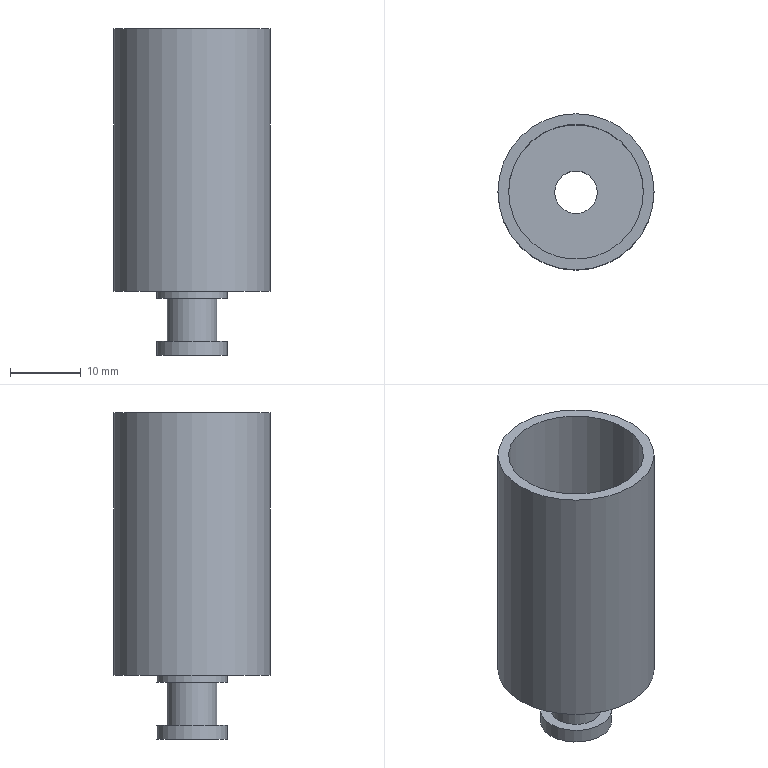Component | NX | PUMP_FLANGE_FITTING | 1 solid | 12 faces | box 22 x 22 x 46 mm | volume 4552 mm3 | plane 6 | cylinder 6 | commonest cylinder face diameters 10 x2 6 x1 7 x1 22 x1 19 x1
STEP:
#1=CARTESIAN_POINT('',(0.,0.,0.));
#2=DIRECTION('',(0.,0.,1.));
#3=DIRECTION('',(1.,0.,0.));
#4=AXIS2_PLACEMENT_3D('',#1,#2,#3);
#5=CARTESIAN_POINT('',(-2.267,-0.01624,77.));
#6=VERTEX_POINT('',#5);
#7=CARTESIAN_POINT('',(-5.267,-0.01624,77.));
#8=DIRECTION('',(0.,0.,1.));
#9=DIRECTION('',(1.,0.,0.));
#10=AXIS2_PLACEMENT_3D('',#7,#8,#9);
#11=CIRCLE('',#10,3.);
#12=CARTESIAN_POINT('',(-5.267,-0.01624,77.));
#13=DIRECTION('',(0.,0.,1.));
#14=DIRECTION('',(1.,0.,0.));
#15=AXIS2_PLACEMENT_3D('',#12,#13,#14);
#16=PLANE('',#15);
#17=CARTESIAN_POINT('',(0.,0.));
#18=DIRECTION('',(1.,0.));
#19=AXIS2_PLACEMENT_2D('',#17,#18);
#20=CIRCLE('',#19,3.);
#21=(GEOMETRIC_REPRESENTATION_CONTEXT(2)PARAMETRIC_REPRESENTATION_CONTEXT()REPRESENTATION_CONTEXT('',''));
#22=DEFINITIONAL_REPRESENTATION('',(#20),#21);
#23=PCURVE('',#16,#22);
#24=CARTESIAN_POINT('',(-5.267,-0.01624,75.));
#25=DIRECTION('',(0.,0.,-1.));
#26=DIRECTION('',(-1.,0.,0.));
#27=AXIS2_PLACEMENT_3D('',#24,#25,#26);
#28=CYLINDRICAL_SURFACE('',#27,3.);
#29=CARTESIAN_POINT('',(9.425,-2.));
#30=DIRECTION('',(-1.,0.));
#31=VECTOR('',#30,1.);
#32=LINE('',#29,#31);
#33=(GEOMETRIC_REPRESENTATION_CONTEXT(2)PARAMETRIC_REPRESENTATION_CONTEXT()REPRESENTATION_CONTEXT('',''));
#34=DEFINITIONAL_REPRESENTATION('',(#32),#33);
#35=PCURVE('',#28,#34);
#36=SURFACE_CURVE('',#11,(#23,#35),.PCURVE_S1.);
#37=EDGE_CURVE('',#6,#6,#36,.T.);
#38=ORIENTED_EDGE('',*,*,#37,.F.);
#39=EDGE_LOOP('',(#38));
#40=FACE_BOUND('',#39,.T.);
#41=CARTESIAN_POINT('',(4.233,-0.01624,77.));
#42=VERTEX_POINT('',#41);
#43=CARTESIAN_POINT('',(-5.267,-0.01624,77.));
#44=DIRECTION('',(0.,0.,1.));
#45=DIRECTION('',(1.,0.,0.));
#46=AXIS2_PLACEMENT_3D('',#43,#44,#45);
#47=CIRCLE('',#46,9.5);
#48=CARTESIAN_POINT('',(0.,0.));
#49=DIRECTION('',(1.,0.));
#50=AXIS2_PLACEMENT_2D('',#48,#49);
#51=CIRCLE('',#50,9.5);
#52=(GEOMETRIC_REPRESENTATION_CONTEXT(2)PARAMETRIC_REPRESENTATION_CONTEXT()REPRESENTATION_CONTEXT('',''));
#53=DEFINITIONAL_REPRESENTATION('',(#51),#52);
#54=PCURVE('',#16,#53);
#55=CARTESIAN_POINT('',(-5.267,-0.01624,111.));
#56=DIRECTION('',(0.,0.,-1.));
#57=DIRECTION('',(-1.,0.,0.));
#58=AXIS2_PLACEMENT_3D('',#55,#56,#57);
#59=CYLINDRICAL_SURFACE('',#58,9.5);
#60=CARTESIAN_POINT('',(9.425,34.));
#61=DIRECTION('',(-1.,0.));
#62=VECTOR('',#61,1.);
#63=LINE('',#60,#62);
#64=(GEOMETRIC_REPRESENTATION_CONTEXT(2)PARAMETRIC_REPRESENTATION_CONTEXT()REPRESENTATION_CONTEXT('',''));
#65=DEFINITIONAL_REPRESENTATION('',(#63),#64);
#66=PCURVE('',#59,#65);
#67=SURFACE_CURVE('',#47,(#54,#66),.PCURVE_S1.);
#68=EDGE_CURVE('',#42,#42,#67,.T.);
#69=ORIENTED_EDGE('',*,*,#68,.T.);
#70=EDGE_LOOP('',(#69));
#71=FACE_BOUND('',#70,.T.);
#72=ADVANCED_FACE('',(#40,#71),#16,.T.);
#73=CARTESIAN_POINT('',(-10.267,-0.01624,73.));
#74=VERTEX_POINT('',#73);
#75=CARTESIAN_POINT('',(-5.267,-0.01624,73.));
#76=DIRECTION('',(0.,0.,-1.));
#77=DIRECTION('',(-1.,0.,0.));
#78=AXIS2_PLACEMENT_3D('',#75,#76,#77);
#79=CIRCLE('',#78,5.);
#80=CARTESIAN_POINT('',(-5.267,-0.01624,75.));
#81=DIRECTION('',(0.,0.,-1.));
#82=DIRECTION('',(-1.,0.,0.));
#83=AXIS2_PLACEMENT_3D('',#80,#81,#82);
#84=CYLINDRICAL_SURFACE('',#83,5.);
#85=CARTESIAN_POINT('',(0.,2.));
#86=DIRECTION('',(1.,0.));
#87=VECTOR('',#86,1.);
#88=LINE('',#85,#87);
#89=(GEOMETRIC_REPRESENTATION_CONTEXT(2)PARAMETRIC_REPRESENTATION_CONTEXT()REPRESENTATION_CONTEXT('',''));
#90=DEFINITIONAL_REPRESENTATION('',(#88),#89);
#91=PCURVE('',#84,#90);
#92=CARTESIAN_POINT('',(-5.267,8.484,73.));
#93=DIRECTION('',(0.,0.,-1.));
#94=DIRECTION('',(-1.,0.,0.));
#95=AXIS2_PLACEMENT_3D('',#92,#93,#94);
#96=PLANE('',#95);
#97=CARTESIAN_POINT('',(0.,-8.5));
#98=DIRECTION('',(1.,0.));
#99=AXIS2_PLACEMENT_2D('',#97,#98);
#100=CIRCLE('',#99,5.);
#101=(GEOMETRIC_REPRESENTATION_CONTEXT(2)PARAMETRIC_REPRESENTATION_CONTEXT()REPRESENTATION_CONTEXT('',''));
#102=DEFINITIONAL_REPRESENTATION('',(#100),#101);
#103=PCURVE('',#96,#102);
#104=SURFACE_CURVE('',#79,(#91,#103),.PCURVE_S1.);
#105=EDGE_CURVE('',#74,#74,#104,.T.);
#106=ORIENTED_EDGE('',*,*,#105,.F.);
#107=CARTESIAN_POINT('',(-10.267,-0.01624,74.));
#108=VERTEX_POINT('',#107);
#109=CARTESIAN_POINT('',(-10.267,-0.01624,74.));
#110=CARTESIAN_POINT('',(-10.267,-0.01624,73.));
#111=B_SPLINE_CURVE_WITH_KNOTS('',1,(#109,#110),.UNSPECIFIED.,.F.,.F.,(2,2),(1.,2.),.PIECEWISE_BEZIER_KNOTS.);
#112=CARTESIAN_POINT('',(0.,0.));
#113=DIRECTION('',(0.,1.));
#114=VECTOR('',#113,1.);
#115=LINE('',#112,#114);
#116=(GEOMETRIC_REPRESENTATION_CONTEXT(2)PARAMETRIC_REPRESENTATION_CONTEXT()REPRESENTATION_CONTEXT('',''));
#117=DEFINITIONAL_REPRESENTATION('',(#115),#116);
#118=PCURVE('',#84,#117);
#119=CARTESIAN_POINT('',(6.283,0.));
#120=DIRECTION('',(0.,1.));
#121=VECTOR('',#120,1.);
#122=LINE('',#119,#121);
#123=(GEOMETRIC_REPRESENTATION_CONTEXT(2)PARAMETRIC_REPRESENTATION_CONTEXT()REPRESENTATION_CONTEXT('',''));
#124=DEFINITIONAL_REPRESENTATION('',(#122),#123);
#125=PCURVE('',#84,#124);
#126=SEAM_CURVE('',#111,(#118,#125),.PCURVE_S1.);
#127=EDGE_CURVE('',#108,#74,#126,.T.);
#128=ORIENTED_EDGE('',*,*,#127,.F.);
#129=CARTESIAN_POINT('',(-0.2668,-0.01624,74.));
#130=VERTEX_POINT('',#129);
#131=CARTESIAN_POINT('',(-5.267,-0.01624,74.));
#132=DIRECTION('',(0.,0.,1.));
#133=DIRECTION('',(1.,0.,0.));
#134=AXIS2_PLACEMENT_3D('',#131,#132,#133);
#135=CIRCLE('',#134,5.);
#136=CARTESIAN_POINT('',(3.142,1.));
#137=DIRECTION('',(-1.,0.));
#138=VECTOR('',#137,1.);
#139=LINE('',#136,#138);
#140=(GEOMETRIC_REPRESENTATION_CONTEXT(2)PARAMETRIC_REPRESENTATION_CONTEXT()REPRESENTATION_CONTEXT('',''));
#141=DEFINITIONAL_REPRESENTATION('',(#139),#140);
#142=PCURVE('',#84,#141);
#143=CARTESIAN_POINT('',(-5.267,-0.01624,74.));
#144=DIRECTION('',(0.,0.,1.));
#145=DIRECTION('',(1.,0.,0.));
#146=AXIS2_PLACEMENT_3D('',#143,#144,#145);
#147=PLANE('',#146);
#148=CARTESIAN_POINT('',(0.,0.));
#149=DIRECTION('',(1.,0.));
#150=AXIS2_PLACEMENT_2D('',#148,#149);
#151=CIRCLE('',#150,5.);
#152=(GEOMETRIC_REPRESENTATION_CONTEXT(2)PARAMETRIC_REPRESENTATION_CONTEXT()REPRESENTATION_CONTEXT('',''));
#153=DEFINITIONAL_REPRESENTATION('',(#151),#152);
#154=PCURVE('',#147,#153);
#155=SURFACE_CURVE('',#135,(#142,#154),.PCURVE_S1.);
#156=EDGE_CURVE('',#130,#108,#155,.T.);
#157=ORIENTED_EDGE('',*,*,#156,.F.);
#158=CARTESIAN_POINT('',(-5.267,-0.01624,74.));
#159=DIRECTION('',(0.,0.,1.));
#160=DIRECTION('',(1.,0.,0.));
#161=AXIS2_PLACEMENT_3D('',#158,#159,#160);
#162=CIRCLE('',#161,5.);
#163=CARTESIAN_POINT('',(9.425,1.));
#164=DIRECTION('',(-1.,0.));
#165=VECTOR('',#164,1.);
#166=LINE('',#163,#165);
#167=(GEOMETRIC_REPRESENTATION_CONTEXT(2)PARAMETRIC_REPRESENTATION_CONTEXT()REPRESENTATION_CONTEXT('',''));
#168=DEFINITIONAL_REPRESENTATION('',(#166),#167);
#169=PCURVE('',#84,#168);
#170=CARTESIAN_POINT('',(0.,0.));
#171=DIRECTION('',(1.,0.));
#172=AXIS2_PLACEMENT_2D('',#170,#171);
#173=CIRCLE('',#172,5.);
#174=(GEOMETRIC_REPRESENTATION_CONTEXT(2)PARAMETRIC_REPRESENTATION_CONTEXT()REPRESENTATION_CONTEXT('',''));
#175=DEFINITIONAL_REPRESENTATION('',(#173),#174);
#176=PCURVE('',#147,#175);
#177=SURFACE_CURVE('',#162,(#169,#176),.PCURVE_S1.);
#178=EDGE_CURVE('',#108,#130,#177,.T.);
#179=ORIENTED_EDGE('',*,*,#178,.F.);
#180=ORIENTED_EDGE('',*,*,#127,.T.);
#181=EDGE_LOOP('',(#106,#128,#157,#179,#180));
#182=FACE_BOUND('',#181,.T.);
#183=ADVANCED_FACE('',(#182),#84,.T.);
#184=CARTESIAN_POINT('',(-0.2668,-0.01624,65.));
#185=VERTEX_POINT('',#184);
#186=CARTESIAN_POINT('',(-5.267,-0.01624,65.));
#187=DIRECTION('',(0.,0.,1.));
#188=DIRECTION('',(1.,0.,0.));
#189=AXIS2_PLACEMENT_3D('',#186,#187,#188);
#190=CIRCLE('',#189,5.);
#191=CARTESIAN_POINT('',(-5.267,-0.01624,75.));
#192=DIRECTION('',(0.,0.,-1.));
#193=DIRECTION('',(-1.,0.,0.));
#194=AXIS2_PLACEMENT_3D('',#191,#192,#193);
#195=CYLINDRICAL_SURFACE('',#194,5.);
#196=CARTESIAN_POINT('',(9.425,10.));
#197=DIRECTION('',(-1.,0.));
#198=VECTOR('',#197,1.);
#199=LINE('',#196,#198);
#200=(GEOMETRIC_REPRESENTATION_CONTEXT(2)PARAMETRIC_REPRESENTATION_CONTEXT()REPRESENTATION_CONTEXT('',''));
#201=DEFINITIONAL_REPRESENTATION('',(#199),#200);
#202=PCURVE('',#195,#201);
#203=CARTESIAN_POINT('',(-5.267,-0.01624,65.));
#204=DIRECTION('',(0.,0.,1.));
#205=DIRECTION('',(1.,0.,0.));
#206=AXIS2_PLACEMENT_3D('',#203,#204,#205);
#207=PLANE('',#206);
#208=CARTESIAN_POINT('',(0.,0.));
#209=DIRECTION('',(1.,0.));
#210=AXIS2_PLACEMENT_2D('',#208,#209);
#211=CIRCLE('',#210,5.);
#212=(GEOMETRIC_REPRESENTATION_CONTEXT(2)PARAMETRIC_REPRESENTATION_CONTEXT()REPRESENTATION_CONTEXT('',''));
#213=DEFINITIONAL_REPRESENTATION('',(#211),#212);
#214=PCURVE('',#207,#213);
#215=SURFACE_CURVE('',#190,(#202,#214),.PCURVE_S1.);
#216=EDGE_CURVE('',#185,#185,#215,.T.);
#217=ORIENTED_EDGE('',*,*,#216,.T.);
#218=CARTESIAN_POINT('',(-0.2668,-0.01624,67.));
#219=VERTEX_POINT('',#218);
#220=CARTESIAN_POINT('',(-0.2668,-0.01624,67.));
#221=CARTESIAN_POINT('',(-0.2668,-0.01624,65.));
#222=B_SPLINE_CURVE_WITH_KNOTS('',1,(#220,#221),.UNSPECIFIED.,.F.,.F.,(2,2),(8.,10.),.PIECEWISE_BEZIER_KNOTS.);
#223=CARTESIAN_POINT('',(3.142,0.));
#224=DIRECTION('',(0.,1.));
#225=VECTOR('',#224,1.);
#226=LINE('',#223,#225);
#227=(GEOMETRIC_REPRESENTATION_CONTEXT(2)PARAMETRIC_REPRESENTATION_CONTEXT()REPRESENTATION_CONTEXT('',''));
#228=DEFINITIONAL_REPRESENTATION('',(#226),#227);
#229=PCURVE('',#195,#228);
#230=CARTESIAN_POINT('',(9.425,0.));
#231=DIRECTION('',(0.,1.));
#232=VECTOR('',#231,1.);
#233=LINE('',#230,#232);
#234=(GEOMETRIC_REPRESENTATION_CONTEXT(2)PARAMETRIC_REPRESENTATION_CONTEXT()REPRESENTATION_CONTEXT('',''));
#235=DEFINITIONAL_REPRESENTATION('',(#233),#234);
#236=PCURVE('',#195,#235);
#237=SEAM_CURVE('',#222,(#229,#236),.PCURVE_S1.);
#238=EDGE_CURVE('',#219,#185,#237,.T.);
#239=ORIENTED_EDGE('',*,*,#238,.F.);
#240=CARTESIAN_POINT('',(-5.267,-0.01624,67.));
#241=DIRECTION('',(0.,0.,1.));
#242=DIRECTION('',(1.,0.,0.));
#243=AXIS2_PLACEMENT_3D('',#240,#241,#242);
#244=CIRCLE('',#243,5.);
#245=CARTESIAN_POINT('',(9.425,8.));
#246=DIRECTION('',(-1.,0.));
#247=VECTOR('',#246,1.);
#248=LINE('',#245,#247);
#249=(GEOMETRIC_REPRESENTATION_CONTEXT(2)PARAMETRIC_REPRESENTATION_CONTEXT()REPRESENTATION_CONTEXT('',''));
#250=DEFINITIONAL_REPRESENTATION('',(#248),#249);
#251=PCURVE('',#195,#250);
#252=CARTESIAN_POINT('',(-5.267,3.484,67.));
#253=DIRECTION('',(0.,0.,1.));
#254=DIRECTION('',(1.,0.,0.));
#255=AXIS2_PLACEMENT_3D('',#252,#253,#254);
#256=PLANE('',#255);
#257=CARTESIAN_POINT('',(0.,-3.5));
#258=DIRECTION('',(1.,0.));
#259=AXIS2_PLACEMENT_2D('',#257,#258);
#260=CIRCLE('',#259,5.);
#261=(GEOMETRIC_REPRESENTATION_CONTEXT(2)PARAMETRIC_REPRESENTATION_CONTEXT()REPRESENTATION_CONTEXT('',''));
#262=DEFINITIONAL_REPRESENTATION('',(#260),#261);
#263=PCURVE('',#256,#262);
#264=SURFACE_CURVE('',#244,(#251,#263),.PCURVE_S1.);
#265=EDGE_CURVE('',#219,#219,#264,.T.);
#266=ORIENTED_EDGE('',*,*,#265,.F.);
#267=ORIENTED_EDGE('',*,*,#238,.T.);
#268=EDGE_LOOP('',(#217,#239,#266,#267));
#269=FACE_BOUND('',#268,.T.);
#270=ADVANCED_FACE('',(#269),#195,.T.);
#271=CARTESIAN_POINT('',(-2.267,-0.01624,65.));
#272=VERTEX_POINT('',#271);
#273=CARTESIAN_POINT('',(-5.267,-0.01624,65.));
#274=DIRECTION('',(0.,0.,1.));
#275=DIRECTION('',(1.,0.,0.));
#276=AXIS2_PLACEMENT_3D('',#273,#274,#275);
#277=CIRCLE('',#276,3.);
#278=CARTESIAN_POINT('',(9.425,10.));
#279=DIRECTION('',(-1.,0.));
#280=VECTOR('',#279,1.);
#281=LINE('',#278,#280);
#282=(GEOMETRIC_REPRESENTATION_CONTEXT(2)PARAMETRIC_REPRESENTATION_CONTEXT()REPRESENTATION_CONTEXT('',''));
#283=DEFINITIONAL_REPRESENTATION('',(#281),#282);
#284=PCURVE('',#28,#283);
#285=CARTESIAN_POINT('',(0.,0.));
#286=DIRECTION('',(1.,0.));
#287=AXIS2_PLACEMENT_2D('',#285,#286);
#288=CIRCLE('',#287,3.);
#289=(GEOMETRIC_REPRESENTATION_CONTEXT(2)PARAMETRIC_REPRESENTATION_CONTEXT()REPRESENTATION_CONTEXT('',''));
#290=DEFINITIONAL_REPRESENTATION('',(#288),#289);
#291=PCURVE('',#207,#290);
#292=SURFACE_CURVE('',#277,(#284,#291),.PCURVE_S1.);
#293=EDGE_CURVE('',#272,#272,#292,.T.);
#294=ORIENTED_EDGE('',*,*,#293,.T.);
#295=CARTESIAN_POINT('',(-2.267,-0.01624,77.));
#296=CARTESIAN_POINT('',(-2.267,-0.01624,65.));
#297=B_SPLINE_CURVE_WITH_KNOTS('',1,(#295,#296),.UNSPECIFIED.,.F.,.F.,(2,2),(-2.,10.),.PIECEWISE_BEZIER_KNOTS.);
#298=CARTESIAN_POINT('',(3.142,0.));
#299=DIRECTION('',(0.,1.));
#300=VECTOR('',#299,1.);
#301=LINE('',#298,#300);
#302=(GEOMETRIC_REPRESENTATION_CONTEXT(2)PARAMETRIC_REPRESENTATION_CONTEXT()REPRESENTATION_CONTEXT('',''));
#303=DEFINITIONAL_REPRESENTATION('',(#301),#302);
#304=PCURVE('',#28,#303);
#305=CARTESIAN_POINT('',(9.425,0.));
#306=DIRECTION('',(0.,1.));
#307=VECTOR('',#306,1.);
#308=LINE('',#305,#307);
#309=(GEOMETRIC_REPRESENTATION_CONTEXT(2)PARAMETRIC_REPRESENTATION_CONTEXT()REPRESENTATION_CONTEXT('',''));
#310=DEFINITIONAL_REPRESENTATION('',(#308),#309);
#311=PCURVE('',#28,#310);
#312=SEAM_CURVE('',#297,(#304,#311),.PCURVE_S1.);
#313=EDGE_CURVE('',#6,#272,#312,.T.);
#314=ORIENTED_EDGE('',*,*,#313,.F.);
#315=ORIENTED_EDGE('',*,*,#37,.F.);
#316=ORIENTED_EDGE('',*,*,#313,.T.);
#317=EDGE_LOOP('',(#294,#314,#315,#316));
#318=FACE_BOUND('',#317,.F.);
#319=ADVANCED_FACE('',(#318),#28,.F.);
#320=ORIENTED_EDGE('',*,*,#216,.F.);
#321=EDGE_LOOP('',(#320));
#322=FACE_BOUND('',#321,.T.);
#323=ORIENTED_EDGE('',*,*,#293,.T.);
#324=EDGE_LOOP('',(#323));
#325=FACE_BOUND('',#324,.T.);
#326=ADVANCED_FACE('',(#322,#325),#207,.F.);
#327=CARTESIAN_POINT('',(-1.767,-0.01624,67.));
#328=VERTEX_POINT('',#327);
#329=CARTESIAN_POINT('',(-5.267,-0.01624,67.));
#330=DIRECTION('',(0.,0.,1.));
#331=DIRECTION('',(1.,0.,0.));
#332=AXIS2_PLACEMENT_3D('',#329,#330,#331);
#333=CIRCLE('',#332,3.5);
#334=CARTESIAN_POINT('',(0.,-3.5));
#335=DIRECTION('',(1.,0.));
#336=AXIS2_PLACEMENT_2D('',#334,#335);
#337=CIRCLE('',#336,3.5);
#338=(GEOMETRIC_REPRESENTATION_CONTEXT(2)PARAMETRIC_REPRESENTATION_CONTEXT()REPRESENTATION_CONTEXT('',''));
#339=DEFINITIONAL_REPRESENTATION('',(#337),#338);
#340=PCURVE('',#256,#339);
#341=CARTESIAN_POINT('',(-5.267,-0.01624,75.));
#342=DIRECTION('',(0.,0.,1.));
#343=DIRECTION('',(1.,0.,0.));
#344=AXIS2_PLACEMENT_3D('',#341,#342,#343);
#345=CYLINDRICAL_SURFACE('',#344,3.5);
#346=CARTESIAN_POINT('',(0.,-8.));
#347=DIRECTION('',(1.,0.));
#348=VECTOR('',#347,1.);
#349=LINE('',#346,#348);
#350=(GEOMETRIC_REPRESENTATION_CONTEXT(2)PARAMETRIC_REPRESENTATION_CONTEXT()REPRESENTATION_CONTEXT('',''));
#351=DEFINITIONAL_REPRESENTATION('',(#349),#350);
#352=PCURVE('',#345,#351);
#353=SURFACE_CURVE('',#333,(#340,#352),.PCURVE_S1.);
#354=EDGE_CURVE('',#328,#328,#353,.T.);
#355=ORIENTED_EDGE('',*,*,#354,.F.);
#356=EDGE_LOOP('',(#355));
#357=FACE_BOUND('',#356,.T.);
#358=ORIENTED_EDGE('',*,*,#265,.T.);
#359=EDGE_LOOP('',(#358));
#360=FACE_BOUND('',#359,.T.);
#361=ADVANCED_FACE('',(#357,#360),#256,.T.);
#362=CARTESIAN_POINT('',(-1.767,-0.01624,73.));
#363=VERTEX_POINT('',#362);
#364=CARTESIAN_POINT('',(-5.267,-0.01624,73.));
#365=DIRECTION('',(0.,0.,1.));
#366=DIRECTION('',(1.,0.,0.));
#367=AXIS2_PLACEMENT_3D('',#364,#365,#366);
#368=CIRCLE('',#367,3.5);
#369=CARTESIAN_POINT('',(-3.5,-8.5));
#370=CARTESIAN_POINT('',(-3.5,-2.438));
#371=CARTESIAN_POINT('',(1.75,-5.469));
#372=CARTESIAN_POINT('',(7.,-8.5));
#373=CARTESIAN_POINT('',(1.75,-11.531));
#374=CARTESIAN_POINT('',(-3.5,-14.562));
#375=CARTESIAN_POINT('',(-3.5,-8.5));
#376=(BOUNDED_CURVE()B_SPLINE_CURVE(2,(#369,#370,#371,#372,#373,#374,#375),.UNSPECIFIED.,.T.,.F.)B_SPLINE_CURVE_WITH_KNOTS((1,2,2,2,2,1),(-2.094,0.,2.094,4.189,6.283,8.378),.UNSPECIFIED.)CURVE()GEOMETRIC_REPRESENTATION_ITEM()RATIONAL_B_SPLINE_CURVE((1.,0.5,1.,0.5,1.,0.5,1.))REPRESENTATION_ITEM(''));
#377=(GEOMETRIC_REPRESENTATION_CONTEXT(2)PARAMETRIC_REPRESENTATION_CONTEXT()REPRESENTATION_CONTEXT('',''));
#378=DEFINITIONAL_REPRESENTATION('',(#376),#377);
#379=PCURVE('',#96,#378);
#380=CARTESIAN_POINT('',(0.,-2.));
#381=DIRECTION('',(1.,0.));
#382=VECTOR('',#381,1.);
#383=LINE('',#380,#382);
#384=(GEOMETRIC_REPRESENTATION_CONTEXT(2)PARAMETRIC_REPRESENTATION_CONTEXT()REPRESENTATION_CONTEXT('',''));
#385=DEFINITIONAL_REPRESENTATION('',(#383),#384);
#386=PCURVE('',#345,#385);
#387=SURFACE_CURVE('',#368,(#379,#386),.PCURVE_S1.);
#388=EDGE_CURVE('',#363,#363,#387,.T.);
#389=ORIENTED_EDGE('',*,*,#388,.T.);
#390=EDGE_LOOP('',(#389));
#391=FACE_BOUND('',#390,.T.);
#392=ORIENTED_EDGE('',*,*,#105,.T.);
#393=EDGE_LOOP('',(#392));
#394=FACE_BOUND('',#393,.T.);
#395=ADVANCED_FACE('',(#391,#394),#96,.T.);
#396=ORIENTED_EDGE('',*,*,#354,.T.);
#397=CARTESIAN_POINT('',(-1.767,-0.01624,67.));
#398=CARTESIAN_POINT('',(-1.767,-0.01624,73.));
#399=B_SPLINE_CURVE_WITH_KNOTS('',1,(#397,#398),.UNSPECIFIED.,.F.,.F.,(2,2),(-8.,-2.),.PIECEWISE_BEZIER_KNOTS.);
#400=CARTESIAN_POINT('',(6.283,0.));
#401=DIRECTION('',(0.,1.));
#402=VECTOR('',#401,1.);
#403=LINE('',#400,#402);
#404=(GEOMETRIC_REPRESENTATION_CONTEXT(2)PARAMETRIC_REPRESENTATION_CONTEXT()REPRESENTATION_CONTEXT('',''));
#405=DEFINITIONAL_REPRESENTATION('',(#403),#404);
#406=PCURVE('',#345,#405);
#407=CARTESIAN_POINT('',(0.,0.));
#408=DIRECTION('',(0.,1.));
#409=VECTOR('',#408,1.);
#410=LINE('',#407,#409);
#411=(GEOMETRIC_REPRESENTATION_CONTEXT(2)PARAMETRIC_REPRESENTATION_CONTEXT()REPRESENTATION_CONTEXT('',''));
#412=DEFINITIONAL_REPRESENTATION('',(#410),#411);
#413=PCURVE('',#345,#412);
#414=SEAM_CURVE('',#399,(#406,#413),.PCURVE_S1.);
#415=EDGE_CURVE('',#328,#363,#414,.T.);
#416=ORIENTED_EDGE('',*,*,#415,.T.);
#417=ORIENTED_EDGE('',*,*,#388,.F.);
#418=ORIENTED_EDGE('',*,*,#415,.F.);
#419=EDGE_LOOP('',(#396,#416,#417,#418));
#420=FACE_BOUND('',#419,.T.);
#421=ADVANCED_FACE('',(#420),#345,.T.);
#422=CARTESIAN_POINT('',(5.733,-0.01624,74.));
#423=VERTEX_POINT('',#422);
#424=CARTESIAN_POINT('',(-5.267,-0.01624,74.));
#425=DIRECTION('',(0.,0.,1.));
#426=DIRECTION('',(1.,0.,0.));
#427=AXIS2_PLACEMENT_3D('',#424,#425,#426);
#428=CIRCLE('',#427,11.);
#429=CARTESIAN_POINT('',(-5.267,-0.01624,74.));
#430=DIRECTION('',(0.,0.,1.));
#431=DIRECTION('',(1.,0.,0.));
#432=AXIS2_PLACEMENT_3D('',#429,#430,#431);
#433=CYLINDRICAL_SURFACE('',#432,11.);
#434=CARTESIAN_POINT('',(0.,0.));
#435=DIRECTION('',(1.,0.));
#436=VECTOR('',#435,1.);
#437=LINE('',#434,#436);
#438=(GEOMETRIC_REPRESENTATION_CONTEXT(2)PARAMETRIC_REPRESENTATION_CONTEXT()REPRESENTATION_CONTEXT('',''));
#439=DEFINITIONAL_REPRESENTATION('',(#437),#438);
#440=PCURVE('',#433,#439);
#441=CARTESIAN_POINT('',(0.,0.));
#442=DIRECTION('',(1.,0.));
#443=AXIS2_PLACEMENT_2D('',#441,#442);
#444=CIRCLE('',#443,11.);
#445=(GEOMETRIC_REPRESENTATION_CONTEXT(2)PARAMETRIC_REPRESENTATION_CONTEXT()REPRESENTATION_CONTEXT('',''));
#446=DEFINITIONAL_REPRESENTATION('',(#444),#445);
#447=PCURVE('',#147,#446);
#448=SURFACE_CURVE('',#428,(#440,#447),.PCURVE_S1.);
#449=EDGE_CURVE('',#423,#423,#448,.T.);
#450=ORIENTED_EDGE('',*,*,#449,.T.);
#451=CARTESIAN_POINT('',(5.733,-0.01624,111.));
#452=VERTEX_POINT('',#451);
#453=CARTESIAN_POINT('',(5.733,-0.01624,74.));
#454=CARTESIAN_POINT('',(5.733,-0.01624,111.));
#455=B_SPLINE_CURVE_WITH_KNOTS('',1,(#453,#454),.UNSPECIFIED.,.F.,.F.,(2,2),(0.,37.),.PIECEWISE_BEZIER_KNOTS.);
#456=CARTESIAN_POINT('',(6.283,0.));
#457=DIRECTION('',(0.,1.));
#458=VECTOR('',#457,1.);
#459=LINE('',#456,#458);
#460=(GEOMETRIC_REPRESENTATION_CONTEXT(2)PARAMETRIC_REPRESENTATION_CONTEXT()REPRESENTATION_CONTEXT('',''));
#461=DEFINITIONAL_REPRESENTATION('',(#459),#460);
#462=PCURVE('',#433,#461);
#463=CARTESIAN_POINT('',(0.,0.));
#464=DIRECTION('',(0.,1.));
#465=VECTOR('',#464,1.);
#466=LINE('',#463,#465);
#467=(GEOMETRIC_REPRESENTATION_CONTEXT(2)PARAMETRIC_REPRESENTATION_CONTEXT()REPRESENTATION_CONTEXT('',''));
#468=DEFINITIONAL_REPRESENTATION('',(#466),#467);
#469=PCURVE('',#433,#468);
#470=SEAM_CURVE('',#455,(#462,#469),.PCURVE_S1.);
#471=EDGE_CURVE('',#423,#452,#470,.T.);
#472=ORIENTED_EDGE('',*,*,#471,.T.);
#473=CARTESIAN_POINT('',(-5.267,-0.01624,111.));
#474=DIRECTION('',(0.,0.,1.));
#475=DIRECTION('',(1.,0.,0.));
#476=AXIS2_PLACEMENT_3D('',#473,#474,#475);
#477=CIRCLE('',#476,11.);
#478=CARTESIAN_POINT('',(0.,37.));
#479=DIRECTION('',(1.,0.));
#480=VECTOR('',#479,1.);
#481=LINE('',#478,#480);
#482=(GEOMETRIC_REPRESENTATION_CONTEXT(2)PARAMETRIC_REPRESENTATION_CONTEXT()REPRESENTATION_CONTEXT('',''));
#483=DEFINITIONAL_REPRESENTATION('',(#481),#482);
#484=PCURVE('',#433,#483);
#485=CARTESIAN_POINT('',(-5.267,-0.01624,111.));
#486=DIRECTION('',(0.,0.,1.));
#487=DIRECTION('',(1.,0.,0.));
#488=AXIS2_PLACEMENT_3D('',#485,#486,#487);
#489=PLANE('',#488);
#490=CARTESIAN_POINT('',(0.,0.));
#491=DIRECTION('',(1.,0.));
#492=AXIS2_PLACEMENT_2D('',#490,#491);
#493=CIRCLE('',#492,11.);
#494=(GEOMETRIC_REPRESENTATION_CONTEXT(2)PARAMETRIC_REPRESENTATION_CONTEXT()REPRESENTATION_CONTEXT('',''));
#495=DEFINITIONAL_REPRESENTATION('',(#493),#494);
#496=PCURVE('',#489,#495);
#497=SURFACE_CURVE('',#477,(#484,#496),.PCURVE_S1.);
#498=EDGE_CURVE('',#452,#452,#497,.T.);
#499=ORIENTED_EDGE('',*,*,#498,.F.);
#500=ORIENTED_EDGE('',*,*,#471,.F.);
#501=EDGE_LOOP('',(#450,#472,#499,#500));
#502=FACE_BOUND('',#501,.T.);
#503=ADVANCED_FACE('',(#502),#433,.T.);
#504=ORIENTED_EDGE('',*,*,#449,.F.);
#505=EDGE_LOOP('',(#504));
#506=FACE_BOUND('',#505,.T.);
#507=ORIENTED_EDGE('',*,*,#156,.T.);
#508=ORIENTED_EDGE('',*,*,#178,.T.);
#509=EDGE_LOOP('',(#507,#508));
#510=FACE_BOUND('',#509,.T.);
#511=ADVANCED_FACE('',(#506,#510),#147,.F.);
#512=CARTESIAN_POINT('',(4.233,-0.01624,111.));
#513=VERTEX_POINT('',#512);
#514=CARTESIAN_POINT('',(-5.267,-0.01624,111.));
#515=DIRECTION('',(0.,0.,1.));
#516=DIRECTION('',(1.,0.,0.));
#517=AXIS2_PLACEMENT_3D('',#514,#515,#516);
#518=CIRCLE('',#517,9.5);
#519=CARTESIAN_POINT('',(9.425,0.));
#520=DIRECTION('',(-1.,0.));
#521=VECTOR('',#520,1.);
#522=LINE('',#519,#521);
#523=(GEOMETRIC_REPRESENTATION_CONTEXT(2)PARAMETRIC_REPRESENTATION_CONTEXT()REPRESENTATION_CONTEXT('',''));
#524=DEFINITIONAL_REPRESENTATION('',(#522),#523);
#525=PCURVE('',#59,#524);
#526=CARTESIAN_POINT('',(0.,0.));
#527=DIRECTION('',(1.,0.));
#528=AXIS2_PLACEMENT_2D('',#526,#527);
#529=CIRCLE('',#528,9.5);
#530=(GEOMETRIC_REPRESENTATION_CONTEXT(2)PARAMETRIC_REPRESENTATION_CONTEXT()REPRESENTATION_CONTEXT('',''));
#531=DEFINITIONAL_REPRESENTATION('',(#529),#530);
#532=PCURVE('',#489,#531);
#533=SURFACE_CURVE('',#518,(#525,#532),.PCURVE_S1.);
#534=EDGE_CURVE('',#513,#513,#533,.T.);
#535=ORIENTED_EDGE('',*,*,#534,.F.);
#536=CARTESIAN_POINT('',(4.233,-0.01624,111.));
#537=CARTESIAN_POINT('',(4.233,-0.01624,77.));
#538=B_SPLINE_CURVE_WITH_KNOTS('',1,(#536,#537),.UNSPECIFIED.,.F.,.F.,(2,2),(0.,34.),.PIECEWISE_BEZIER_KNOTS.);
#539=CARTESIAN_POINT('',(9.425,0.));
#540=DIRECTION('',(0.,1.));
#541=VECTOR('',#540,1.);
#542=LINE('',#539,#541);
#543=(GEOMETRIC_REPRESENTATION_CONTEXT(2)PARAMETRIC_REPRESENTATION_CONTEXT()REPRESENTATION_CONTEXT('',''));
#544=DEFINITIONAL_REPRESENTATION('',(#542),#543);
#545=PCURVE('',#59,#544);
#546=CARTESIAN_POINT('',(3.142,0.));
#547=DIRECTION('',(0.,1.));
#548=VECTOR('',#547,1.);
#549=LINE('',#546,#548);
#550=(GEOMETRIC_REPRESENTATION_CONTEXT(2)PARAMETRIC_REPRESENTATION_CONTEXT()REPRESENTATION_CONTEXT('',''));
#551=DEFINITIONAL_REPRESENTATION('',(#549),#550);
#552=PCURVE('',#59,#551);
#553=SEAM_CURVE('',#538,(#545,#552),.PCURVE_S1.);
#554=EDGE_CURVE('',#513,#42,#553,.T.);
#555=ORIENTED_EDGE('',*,*,#554,.T.);
#556=ORIENTED_EDGE('',*,*,#68,.T.);
#557=ORIENTED_EDGE('',*,*,#554,.F.);
#558=EDGE_LOOP('',(#535,#555,#556,#557));
#559=FACE_BOUND('',#558,.F.);
#560=ADVANCED_FACE('',(#559),#59,.F.);
#561=ORIENTED_EDGE('',*,*,#498,.T.);
#562=EDGE_LOOP('',(#561));
#563=FACE_BOUND('',#562,.T.);
#564=ORIENTED_EDGE('',*,*,#534,.F.);
#565=EDGE_LOOP('',(#564));
#566=FACE_BOUND('',#565,.T.);
#567=ADVANCED_FACE('',(#563,#566),#489,.T.);
#568=CLOSED_SHELL('',(#72,#183,#270,#319,#326,#361,#395,#421,#503,#511,#560,#567));
#569=MANIFOLD_SOLID_BREP('',#568);
#570=(LENGTH_UNIT()NAMED_UNIT(*)SI_UNIT(.MILLI.,.METRE.));
#571=UNCERTAINTY_MEASURE_WITH_UNIT(LENGTH_MEASURE(0.00001),#570,'','');
#572=(NAMED_UNIT(*)PLANE_ANGLE_UNIT()SI_UNIT($,.RADIAN.));
#573=(NAMED_UNIT(*)SI_UNIT($,.STERADIAN.)SOLID_ANGLE_UNIT());
#574=(GEOMETRIC_REPRESENTATION_CONTEXT(3)GLOBAL_UNCERTAINTY_ASSIGNED_CONTEXT((#571))GLOBAL_UNIT_ASSIGNED_CONTEXT((#570,#572,#573))REPRESENTATION_CONTEXT('',''));
#575=ADVANCED_BREP_SHAPE_REPRESENTATION('',(#4,#569),#574);